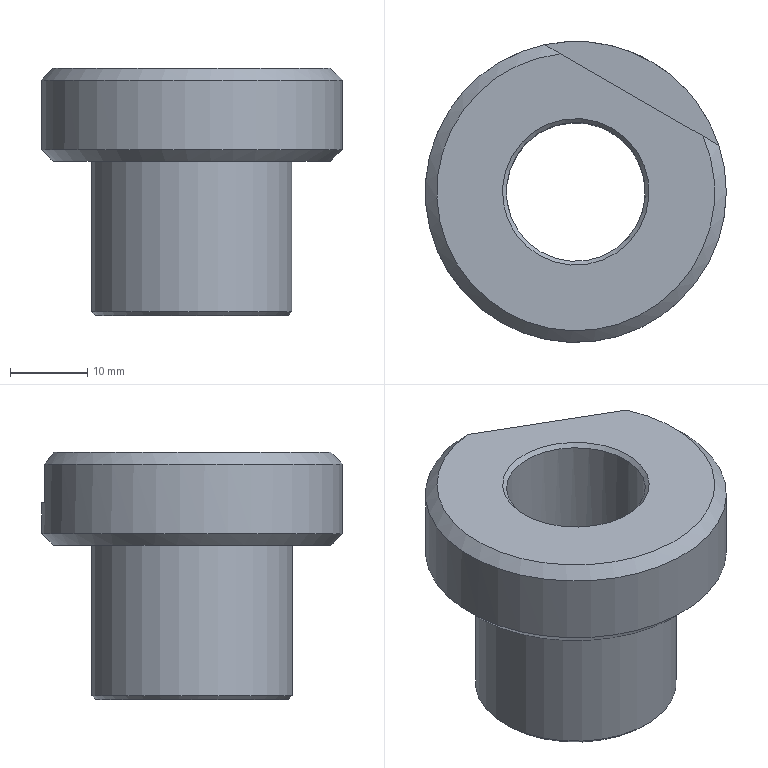Component | NX | DRILL_BUSH | 1 solid | 13 faces | box 39 x 39 x 32 mm | volume 15966 mm3 | plane 5 | cone 5 | cylinder 3 | commonest cylinder face diameters 26 x1 39 x1 18 x1
STEP:
#1=CARTESIAN_POINT('',(0.,0.,0.));
#2=DIRECTION('',(0.,0.,1.));
#3=DIRECTION('',(1.,0.,0.));
#4=AXIS2_PLACEMENT_3D('',#1,#2,#3);
#5=CARTESIAN_POINT('',(-46.25,-80.107,180.));
#6=VERTEX_POINT('',#5);
#7=CARTESIAN_POINT('',(-40.,-69.282,180.));
#8=DIRECTION('',(0.,0.,-1.));
#9=DIRECTION('',(-0.5,-0.866,0.));
#10=AXIS2_PLACEMENT_3D('',#7,#8,#9);
#11=CIRCLE('',#10,12.5);
#12=CARTESIAN_POINT('',(-40.,-69.282,180.));
#13=DIRECTION('',(0.,0.,-1.));
#14=DIRECTION('',(-0.5,-0.866,0.));
#15=AXIS2_PLACEMENT_3D('',#12,#13,#14);
#16=PLANE('',#15);
#17=CARTESIAN_POINT('',(0.,0.));
#18=DIRECTION('',(1.,0.));
#19=AXIS2_PLACEMENT_2D('',#17,#18);
#20=CIRCLE('',#19,12.5);
#21=(GEOMETRIC_REPRESENTATION_CONTEXT(2)PARAMETRIC_REPRESENTATION_CONTEXT()REPRESENTATION_CONTEXT('',''));
#22=DEFINITIONAL_REPRESENTATION('',(#20),#21);
#23=PCURVE('',#16,#22);
#24=CARTESIAN_POINT('',(-40.,-69.282,180.5));
#25=DIRECTION('',(0.,0.,1.));
#26=DIRECTION('',(0.5,0.866,0.));
#27=AXIS2_PLACEMENT_3D('',#24,#25,#26);
#28=CONICAL_SURFACE('',#27,13.,0.7854);
#29=CARTESIAN_POINT('',(9.425,-0.5));
#30=DIRECTION('',(-1.,0.));
#31=VECTOR('',#30,1.);
#32=LINE('',#29,#31);
#33=(GEOMETRIC_REPRESENTATION_CONTEXT(2)PARAMETRIC_REPRESENTATION_CONTEXT()REPRESENTATION_CONTEXT('',''));
#34=DEFINITIONAL_REPRESENTATION('',(#32),#33);
#35=PCURVE('',#28,#34);
#36=SURFACE_CURVE('',#11,(#23,#35),.PCURVE_S1.);
#37=EDGE_CURVE('',#6,#6,#36,.T.);
#38=ORIENTED_EDGE('',*,*,#37,.T.);
#39=EDGE_LOOP('',(#38));
#40=FACE_BOUND('',#39,.T.);
#41=CARTESIAN_POINT('',(-44.75,-77.509,180.));
#42=VERTEX_POINT('',#41);
#43=CARTESIAN_POINT('',(-40.,-69.282,180.));
#44=DIRECTION('',(0.,0.,1.));
#45=DIRECTION('',(-0.5,-0.866,0.));
#46=AXIS2_PLACEMENT_3D('',#43,#44,#45);
#47=CIRCLE('',#46,9.5);
#48=CARTESIAN_POINT('',(9.5,0.));
#49=CARTESIAN_POINT('',(9.5,-16.454));
#50=CARTESIAN_POINT('',(-4.75,-8.227));
#51=CARTESIAN_POINT('',(-19.,-0.));
#52=CARTESIAN_POINT('',(-4.75,8.227));
#53=CARTESIAN_POINT('',(9.5,16.454));
#54=CARTESIAN_POINT('',(9.5,0.));
#55=(BOUNDED_CURVE()B_SPLINE_CURVE(2,(#48,#49,#50,#51,#52,#53,#54),.UNSPECIFIED.,.T.,.F.)B_SPLINE_CURVE_WITH_KNOTS((1,2,2,2,2,1),(-2.094,0.,2.094,4.189,6.283,8.378),.UNSPECIFIED.)CURVE()GEOMETRIC_REPRESENTATION_ITEM()RATIONAL_B_SPLINE_CURVE((1.,0.5,1.,0.5,1.,0.5,1.))REPRESENTATION_ITEM(''));
#56=(GEOMETRIC_REPRESENTATION_CONTEXT(2)PARAMETRIC_REPRESENTATION_CONTEXT()REPRESENTATION_CONTEXT('',''));
#57=DEFINITIONAL_REPRESENTATION('',(#55),#56);
#58=PCURVE('',#16,#57);
#59=CARTESIAN_POINT('',(-40.,-69.282,180.5));
#60=DIRECTION('',(0.,0.,-1.));
#61=DIRECTION('',(-0.5,-0.866,0.));
#62=AXIS2_PLACEMENT_3D('',#59,#60,#61);
#63=CONICAL_SURFACE('',#62,9.,0.7854);
#64=CARTESIAN_POINT('',(6.283,0.5));
#65=DIRECTION('',(-1.,0.));
#66=VECTOR('',#65,1.);
#67=LINE('',#64,#66);
#68=(GEOMETRIC_REPRESENTATION_CONTEXT(2)PARAMETRIC_REPRESENTATION_CONTEXT()REPRESENTATION_CONTEXT('',''));
#69=DEFINITIONAL_REPRESENTATION('',(#67),#68);
#70=PCURVE('',#63,#69);
#71=SURFACE_CURVE('',#47,(#58,#70),.PCURVE_S1.);
#72=EDGE_CURVE('',#42,#42,#71,.T.);
#73=ORIENTED_EDGE('',*,*,#72,.T.);
#74=EDGE_LOOP('',(#73));
#75=FACE_BOUND('',#74,.T.);
#76=ADVANCED_FACE('',(#40,#75),#16,.T.);
#77=CARTESIAN_POINT('',(-46.5,-80.54,180.5));
#78=VERTEX_POINT('',#77);
#79=CARTESIAN_POINT('',(-40.,-69.282,180.5));
#80=DIRECTION('',(0.,0.,1.));
#81=DIRECTION('',(-0.5,-0.866,0.));
#82=AXIS2_PLACEMENT_3D('',#79,#80,#81);
#83=CIRCLE('',#82,13.);
#84=CARTESIAN_POINT('',(-40.,-69.282,180.));
#85=DIRECTION('',(0.,0.,1.));
#86=DIRECTION('',(0.5,0.866,0.));
#87=AXIS2_PLACEMENT_3D('',#84,#85,#86);
#88=CYLINDRICAL_SURFACE('',#87,13.);
#89=CARTESIAN_POINT('',(3.142,0.5));
#90=DIRECTION('',(1.,0.));
#91=VECTOR('',#90,1.);
#92=LINE('',#89,#91);
#93=(GEOMETRIC_REPRESENTATION_CONTEXT(2)PARAMETRIC_REPRESENTATION_CONTEXT()REPRESENTATION_CONTEXT('',''));
#94=DEFINITIONAL_REPRESENTATION('',(#92),#93);
#95=PCURVE('',#88,#94);
#96=CARTESIAN_POINT('',(3.142,0.));
#97=DIRECTION('',(1.,0.));
#98=VECTOR('',#97,1.);
#99=LINE('',#96,#98);
#100=(GEOMETRIC_REPRESENTATION_CONTEXT(2)PARAMETRIC_REPRESENTATION_CONTEXT()REPRESENTATION_CONTEXT('',''));
#101=DEFINITIONAL_REPRESENTATION('',(#99),#100);
#102=PCURVE('',#28,#101);
#103=SURFACE_CURVE('',#83,(#95,#102),.PCURVE_S1.);
#104=EDGE_CURVE('',#78,#78,#103,.T.);
#105=ORIENTED_EDGE('',*,*,#104,.T.);
#106=CARTESIAN_POINT('',(-46.5,-80.54,200.));
#107=VERTEX_POINT('',#106);
#108=CARTESIAN_POINT('',(-46.5,-80.54,180.5));
#109=CARTESIAN_POINT('',(-46.5,-80.54,200.));
#110=B_SPLINE_CURVE_WITH_KNOTS('',1,(#108,#109),.UNSPECIFIED.,.F.,.F.,(2,2),(0.5,20.),.PIECEWISE_BEZIER_KNOTS.);
#111=CARTESIAN_POINT('',(9.425,0.));
#112=DIRECTION('',(0.,1.));
#113=VECTOR('',#112,1.);
#114=LINE('',#111,#113);
#115=(GEOMETRIC_REPRESENTATION_CONTEXT(2)PARAMETRIC_REPRESENTATION_CONTEXT()REPRESENTATION_CONTEXT('',''));
#116=DEFINITIONAL_REPRESENTATION('',(#114),#115);
#117=PCURVE('',#88,#116);
#118=CARTESIAN_POINT('',(3.142,0.));
#119=DIRECTION('',(0.,1.));
#120=VECTOR('',#119,1.);
#121=LINE('',#118,#120);
#122=(GEOMETRIC_REPRESENTATION_CONTEXT(2)PARAMETRIC_REPRESENTATION_CONTEXT()REPRESENTATION_CONTEXT('',''));
#123=DEFINITIONAL_REPRESENTATION('',(#121),#122);
#124=PCURVE('',#88,#123);
#125=SEAM_CURVE('',#110,(#117,#124),.PCURVE_S1.);
#126=EDGE_CURVE('',#78,#107,#125,.T.);
#127=ORIENTED_EDGE('',*,*,#126,.T.);
#128=CARTESIAN_POINT('',(-40.,-69.282,200.));
#129=DIRECTION('',(0.,0.,1.));
#130=DIRECTION('',(-0.5,-0.866,0.));
#131=AXIS2_PLACEMENT_3D('',#128,#129,#130);
#132=CIRCLE('',#131,13.);
#133=CARTESIAN_POINT('',(3.142,20.));
#134=DIRECTION('',(1.,0.));
#135=VECTOR('',#134,1.);
#136=LINE('',#133,#135);
#137=(GEOMETRIC_REPRESENTATION_CONTEXT(2)PARAMETRIC_REPRESENTATION_CONTEXT()REPRESENTATION_CONTEXT('',''));
#138=DEFINITIONAL_REPRESENTATION('',(#136),#137);
#139=PCURVE('',#88,#138);
#140=CARTESIAN_POINT('',(-40.,-69.282,200.));
#141=DIRECTION('',(0.,0.,-1.));
#142=DIRECTION('',(-0.5,-0.866,0.));
#143=AXIS2_PLACEMENT_3D('',#140,#141,#142);
#144=PLANE('',#143);
#145=CARTESIAN_POINT('',(13.,0.));
#146=CARTESIAN_POINT('',(13.,-22.517));
#147=CARTESIAN_POINT('',(-6.5,-11.258));
#148=CARTESIAN_POINT('',(-26.,-0.));
#149=CARTESIAN_POINT('',(-6.5,11.258));
#150=CARTESIAN_POINT('',(13.,22.517));
#151=CARTESIAN_POINT('',(13.,0.));
#152=(BOUNDED_CURVE()B_SPLINE_CURVE(2,(#145,#146,#147,#148,#149,#150,#151),.UNSPECIFIED.,.T.,.F.)B_SPLINE_CURVE_WITH_KNOTS((1,2,2,2,2,1),(-2.094,0.,2.094,4.189,6.283,8.378),.UNSPECIFIED.)CURVE()GEOMETRIC_REPRESENTATION_ITEM()RATIONAL_B_SPLINE_CURVE((1.,0.5,1.,0.5,1.,0.5,1.))REPRESENTATION_ITEM(''));
#153=(GEOMETRIC_REPRESENTATION_CONTEXT(2)PARAMETRIC_REPRESENTATION_CONTEXT()REPRESENTATION_CONTEXT('',''));
#154=DEFINITIONAL_REPRESENTATION('',(#152),#153);
#155=PCURVE('',#144,#154);
#156=SURFACE_CURVE('',#132,(#139,#155),.PCURVE_S1.);
#157=EDGE_CURVE('',#107,#107,#156,.T.);
#158=ORIENTED_EDGE('',*,*,#157,.F.);
#159=ORIENTED_EDGE('',*,*,#126,.F.);
#160=EDGE_LOOP('',(#105,#127,#158,#159));
#161=FACE_BOUND('',#160,.T.);
#162=ADVANCED_FACE('',(#161),#88,.T.);
#163=CARTESIAN_POINT('',(-35.25,-61.055,212.));
#164=VERTEX_POINT('',#163);
#165=CARTESIAN_POINT('',(-40.,-69.282,212.));
#166=DIRECTION('',(0.,0.,-1.));
#167=DIRECTION('',(0.5,0.866,0.));
#168=AXIS2_PLACEMENT_3D('',#165,#166,#167);
#169=CIRCLE('',#168,9.5);
#170=CARTESIAN_POINT('',(-40.,-69.282,212.));
#171=DIRECTION('',(0.,0.,1.));
#172=DIRECTION('',(0.5,0.866,0.));
#173=AXIS2_PLACEMENT_3D('',#170,#171,#172);
#174=PLANE('',#173);
#175=CARTESIAN_POINT('',(9.5,0.));
#176=CARTESIAN_POINT('',(9.5,-16.454));
#177=CARTESIAN_POINT('',(-4.75,-8.227));
#178=CARTESIAN_POINT('',(-19.,-0.));
#179=CARTESIAN_POINT('',(-4.75,8.227));
#180=CARTESIAN_POINT('',(9.5,16.454));
#181=CARTESIAN_POINT('',(9.5,0.));
#182=(BOUNDED_CURVE()B_SPLINE_CURVE(2,(#175,#176,#177,#178,#179,#180,#181),.UNSPECIFIED.,.T.,.F.)B_SPLINE_CURVE_WITH_KNOTS((1,2,2,2,2,1),(-2.094,0.,2.094,4.189,6.283,8.378),.UNSPECIFIED.)CURVE()GEOMETRIC_REPRESENTATION_ITEM()RATIONAL_B_SPLINE_CURVE((1.,0.5,1.,0.5,1.,0.5,1.))REPRESENTATION_ITEM(''));
#183=(GEOMETRIC_REPRESENTATION_CONTEXT(2)PARAMETRIC_REPRESENTATION_CONTEXT()REPRESENTATION_CONTEXT('',''));
#184=DEFINITIONAL_REPRESENTATION('',(#182),#183);
#185=PCURVE('',#174,#184);
#186=CARTESIAN_POINT('',(-40.,-69.282,212.));
#187=DIRECTION('',(0.,0.,1.));
#188=DIRECTION('',(0.5,0.866,0.));
#189=AXIS2_PLACEMENT_3D('',#186,#187,#188);
#190=CONICAL_SURFACE('',#189,9.5,0.7854);
#191=CARTESIAN_POINT('',(6.283,0.));
#192=DIRECTION('',(-1.,0.));
#193=VECTOR('',#192,1.);
#194=LINE('',#191,#193);
#195=(GEOMETRIC_REPRESENTATION_CONTEXT(2)PARAMETRIC_REPRESENTATION_CONTEXT()REPRESENTATION_CONTEXT('',''));
#196=DEFINITIONAL_REPRESENTATION('',(#194),#195);
#197=PCURVE('',#190,#196);
#198=SURFACE_CURVE('',#169,(#185,#197),.PCURVE_S1.);
#199=EDGE_CURVE('',#164,#164,#198,.T.);
#200=ORIENTED_EDGE('',*,*,#199,.T.);
#201=EDGE_LOOP('',(#200));
#202=FACE_BOUND('',#201,.T.);
#203=CARTESIAN_POINT('',(-41.986,-51.392,212.));
#204=VERTEX_POINT('',#203);
#205=CARTESIAN_POINT('',(-23.514,-62.057,212.));
#206=VERTEX_POINT('',#205);
#207=CARTESIAN_POINT('',(-52.669,-45.225,212.));
#208=DIRECTION('',(0.866,-0.5,0.));
#209=VECTOR('',#208,1.);
#210=LINE('',#207,#209);
#211=CARTESIAN_POINT('',(14.5,23.));
#212=DIRECTION('',(0.,-1.));
#213=VECTOR('',#212,1.);
#214=LINE('',#211,#213);
#215=(GEOMETRIC_REPRESENTATION_CONTEXT(2)PARAMETRIC_REPRESENTATION_CONTEXT()REPRESENTATION_CONTEXT('',''));
#216=DEFINITIONAL_REPRESENTATION('',(#214),#215);
#217=PCURVE('',#174,#216);
#218=CARTESIAN_POINT('',(-52.669,-45.225,205.5));
#219=DIRECTION('',(-0.5,-0.866,0.));
#220=DIRECTION('',(0.866,-0.5,0.));
#221=AXIS2_PLACEMENT_3D('',#218,#219,#220);
#222=PLANE('',#221);
#223=CARTESIAN_POINT('',(0.,6.5));
#224=DIRECTION('',(1.,0.));
#225=VECTOR('',#224,1.);
#226=LINE('',#223,#225);
#227=(GEOMETRIC_REPRESENTATION_CONTEXT(2)PARAMETRIC_REPRESENTATION_CONTEXT()REPRESENTATION_CONTEXT('',''));
#228=DEFINITIONAL_REPRESENTATION('',(#226),#227);
#229=PCURVE('',#222,#228);
#230=SURFACE_CURVE('',#210,(#217,#229),.PCURVE_S1.);
#231=EDGE_CURVE('',#204,#206,#230,.T.);
#232=ORIENTED_EDGE('',*,*,#231,.F.);
#233=CARTESIAN_POINT('',(-40.,-69.282,212.));
#234=DIRECTION('',(0.,0.,1.));
#235=DIRECTION('',(0.5,0.866,0.));
#236=AXIS2_PLACEMENT_3D('',#233,#234,#235);
#237=CIRCLE('',#236,18.);
#238=CARTESIAN_POINT('',(0.,0.));
#239=DIRECTION('',(1.,0.));
#240=AXIS2_PLACEMENT_2D('',#238,#239);
#241=CIRCLE('',#240,18.);
#242=(GEOMETRIC_REPRESENTATION_CONTEXT(2)PARAMETRIC_REPRESENTATION_CONTEXT()REPRESENTATION_CONTEXT('',''));
#243=DEFINITIONAL_REPRESENTATION('',(#241),#242);
#244=PCURVE('',#174,#243);
#245=CARTESIAN_POINT('',(-40.,-69.282,210.5));
#246=DIRECTION('',(0.,0.,-1.));
#247=DIRECTION('',(-0.5,-0.866,0.));
#248=AXIS2_PLACEMENT_3D('',#245,#246,#247);
#249=CONICAL_SURFACE('',#248,19.5,0.7854);
#250=CARTESIAN_POINT('',(9.425,-1.5));
#251=DIRECTION('',(-1.,0.));
#252=VECTOR('',#251,1.);
#253=LINE('',#250,#252);
#254=(GEOMETRIC_REPRESENTATION_CONTEXT(2)PARAMETRIC_REPRESENTATION_CONTEXT()REPRESENTATION_CONTEXT('',''));
#255=DEFINITIONAL_REPRESENTATION('',(#253),#254);
#256=PCURVE('',#249,#255);
#257=SURFACE_CURVE('',#237,(#244,#256),.PCURVE_S1.);
#258=EDGE_CURVE('',#204,#206,#257,.T.);
#259=ORIENTED_EDGE('',*,*,#258,.T.);
#260=EDGE_LOOP('',(#232,#259));
#261=FACE_BOUND('',#260,.T.);
#262=ADVANCED_FACE('',(#202,#261),#174,.T.);
#263=CARTESIAN_POINT('',(-49.,-84.87,200.));
#264=VERTEX_POINT('',#263);
#265=CARTESIAN_POINT('',(-40.,-69.282,200.));
#266=DIRECTION('',(0.,0.,-1.));
#267=DIRECTION('',(-0.5,-0.866,0.));
#268=AXIS2_PLACEMENT_3D('',#265,#266,#267);
#269=CIRCLE('',#268,18.);
#270=CARTESIAN_POINT('',(0.,0.));
#271=DIRECTION('',(1.,0.));
#272=AXIS2_PLACEMENT_2D('',#270,#271);
#273=CIRCLE('',#272,18.);
#274=(GEOMETRIC_REPRESENTATION_CONTEXT(2)PARAMETRIC_REPRESENTATION_CONTEXT()REPRESENTATION_CONTEXT('',''));
#275=DEFINITIONAL_REPRESENTATION('',(#273),#274);
#276=PCURVE('',#144,#275);
#277=CARTESIAN_POINT('',(-40.,-69.282,201.5));
#278=DIRECTION('',(0.,0.,1.));
#279=DIRECTION('',(0.5,0.866,0.));
#280=AXIS2_PLACEMENT_3D('',#277,#278,#279);
#281=CONICAL_SURFACE('',#280,19.5,0.7854);
#282=CARTESIAN_POINT('',(9.425,-1.5));
#283=DIRECTION('',(-1.,0.));
#284=VECTOR('',#283,1.);
#285=LINE('',#282,#284);
#286=(GEOMETRIC_REPRESENTATION_CONTEXT(2)PARAMETRIC_REPRESENTATION_CONTEXT()REPRESENTATION_CONTEXT('',''));
#287=DEFINITIONAL_REPRESENTATION('',(#285),#286);
#288=PCURVE('',#281,#287);
#289=SURFACE_CURVE('',#269,(#276,#288),.PCURVE_S1.);
#290=EDGE_CURVE('',#264,#264,#289,.T.);
#291=ORIENTED_EDGE('',*,*,#290,.T.);
#292=EDGE_LOOP('',(#291));
#293=FACE_BOUND('',#292,.T.);
#294=ORIENTED_EDGE('',*,*,#157,.T.);
#295=EDGE_LOOP('',(#294));
#296=FACE_BOUND('',#295,.T.);
#297=ADVANCED_FACE('',(#293,#296),#144,.T.);
#298=CARTESIAN_POINT('',(-49.75,-86.17,201.5));
#299=VERTEX_POINT('',#298);
#300=CARTESIAN_POINT('',(-21.458,-63.244,201.5));
#301=VERTEX_POINT('',#300);
#302=CARTESIAN_POINT('',(-40.,-69.282,201.5));
#303=DIRECTION('',(0.,0.,1.));
#304=DIRECTION('',(-0.5,-0.866,0.));
#305=AXIS2_PLACEMENT_3D('',#302,#303,#304);
#306=CIRCLE('',#305,19.5);
#307=CARTESIAN_POINT('',(-40.,-69.282,200.));
#308=DIRECTION('',(0.,0.,1.));
#309=DIRECTION('',(0.5,0.866,0.));
#310=AXIS2_PLACEMENT_3D('',#307,#308,#309);
#311=CYLINDRICAL_SURFACE('',#310,19.5);
#312=CARTESIAN_POINT('',(9.425,1.5));
#313=DIRECTION('',(1.,0.));
#314=VECTOR('',#313,1.);
#315=LINE('',#312,#314);
#316=(GEOMETRIC_REPRESENTATION_CONTEXT(2)PARAMETRIC_REPRESENTATION_CONTEXT()REPRESENTATION_CONTEXT('',''));
#317=DEFINITIONAL_REPRESENTATION('',(#315),#316);
#318=PCURVE('',#311,#317);
#319=CARTESIAN_POINT('',(3.142,0.));
#320=DIRECTION('',(1.,-0.));
#321=VECTOR('',#320,1.);
#322=LINE('',#319,#321);
#323=(GEOMETRIC_REPRESENTATION_CONTEXT(2)PARAMETRIC_REPRESENTATION_CONTEXT()REPRESENTATION_CONTEXT('',''));
#324=DEFINITIONAL_REPRESENTATION('',(#322),#323);
#325=PCURVE('',#281,#324);
#326=SURFACE_CURVE('',#306,(#318,#325),.PCURVE_S1.);
#327=EDGE_CURVE('',#299,#301,#326,.T.);
#328=ORIENTED_EDGE('',*,*,#327,.T.);
#329=CARTESIAN_POINT('',(-21.458,-63.244,205.5));
#330=VERTEX_POINT('',#329);
#331=CARTESIAN_POINT('',(-21.458,-63.244,201.5));
#332=CARTESIAN_POINT('',(-21.458,-63.244,205.5));
#333=B_SPLINE_CURVE_WITH_KNOTS('',1,(#331,#332),.UNSPECIFIED.,.F.,.F.,(2,2),(1.5,5.5),.PIECEWISE_BEZIER_KNOTS.);
#334=CARTESIAN_POINT('',(11.834,0.));
#335=DIRECTION('',(0.,1.));
#336=VECTOR('',#335,1.);
#337=LINE('',#334,#336);
#338=(GEOMETRIC_REPRESENTATION_CONTEXT(2)PARAMETRIC_REPRESENTATION_CONTEXT()REPRESENTATION_CONTEXT('',''));
#339=DEFINITIONAL_REPRESENTATION('',(#337),#338);
#340=PCURVE('',#311,#339);
#341=CARTESIAN_POINT('',(5.551,0.));
#342=DIRECTION('',(0.,1.));
#343=VECTOR('',#342,1.);
#344=LINE('',#341,#343);
#345=(GEOMETRIC_REPRESENTATION_CONTEXT(2)PARAMETRIC_REPRESENTATION_CONTEXT()REPRESENTATION_CONTEXT('',''));
#346=DEFINITIONAL_REPRESENTATION('',(#344),#345);
#347=PCURVE('',#311,#346);
#348=SEAM_CURVE('',#333,(#340,#347),.PCURVE_S1.);
#349=EDGE_CURVE('',#301,#330,#348,.T.);
#350=ORIENTED_EDGE('',*,*,#349,.T.);
#351=CARTESIAN_POINT('',(-21.458,-63.244,210.5));
#352=VERTEX_POINT('',#351);
#353=CARTESIAN_POINT('',(-21.458,-63.244,200.));
#354=DIRECTION('',(0.,0.,-1.));
#355=VECTOR('',#354,1.);
#356=LINE('',#353,#355);
#357=CARTESIAN_POINT('',(11.834,0.));
#358=DIRECTION('',(0.,-1.));
#359=VECTOR('',#358,1.);
#360=LINE('',#357,#359);
#361=(GEOMETRIC_REPRESENTATION_CONTEXT(2)PARAMETRIC_REPRESENTATION_CONTEXT()REPRESENTATION_CONTEXT('',''));
#362=DEFINITIONAL_REPRESENTATION('',(#360),#361);
#363=PCURVE('',#311,#362);
#364=CARTESIAN_POINT('',(36.038,-5.5));
#365=DIRECTION('',(0.,-1.));
#366=VECTOR('',#365,1.);
#367=LINE('',#364,#366);
#368=(GEOMETRIC_REPRESENTATION_CONTEXT(2)PARAMETRIC_REPRESENTATION_CONTEXT()REPRESENTATION_CONTEXT('',''));
#369=DEFINITIONAL_REPRESENTATION('',(#367),#368);
#370=PCURVE('',#222,#369);
#371=SURFACE_CURVE('',#356,(#363,#370),.PCURVE_S1.);
#372=EDGE_CURVE('',#352,#330,#371,.T.);
#373=ORIENTED_EDGE('',*,*,#372,.F.);
#374=CARTESIAN_POINT('',(-44.042,-50.205,210.5));
#375=VERTEX_POINT('',#374);
#376=CARTESIAN_POINT('',(-40.,-69.282,210.5));
#377=DIRECTION('',(0.,0.,-1.));
#378=DIRECTION('',(0.5,0.866,0.));
#379=AXIS2_PLACEMENT_3D('',#376,#377,#378);
#380=CIRCLE('',#379,19.5);
#381=CARTESIAN_POINT('',(12.566,10.5));
#382=DIRECTION('',(-1.,0.));
#383=VECTOR('',#382,1.);
#384=LINE('',#381,#383);
#385=(GEOMETRIC_REPRESENTATION_CONTEXT(2)PARAMETRIC_REPRESENTATION_CONTEXT()REPRESENTATION_CONTEXT('',''));
#386=DEFINITIONAL_REPRESENTATION('',(#384),#385);
#387=PCURVE('',#311,#386);
#388=CARTESIAN_POINT('',(3.142,0.));
#389=DIRECTION('',(1.,-0.));
#390=VECTOR('',#389,1.);
#391=LINE('',#388,#390);
#392=(GEOMETRIC_REPRESENTATION_CONTEXT(2)PARAMETRIC_REPRESENTATION_CONTEXT()REPRESENTATION_CONTEXT('',''));
#393=DEFINITIONAL_REPRESENTATION('',(#391),#392);
#394=PCURVE('',#249,#393);
#395=SURFACE_CURVE('',#380,(#387,#394),.PCURVE_S1.);
#396=EDGE_CURVE('',#352,#375,#395,.T.);
#397=ORIENTED_EDGE('',*,*,#396,.T.);
#398=CARTESIAN_POINT('',(-44.042,-50.205,205.5));
#399=VERTEX_POINT('',#398);
#400=CARTESIAN_POINT('',(-44.042,-50.205,200.));
#401=DIRECTION('',(0.,0.,1.));
#402=VECTOR('',#401,1.);
#403=LINE('',#400,#402);
#404=CARTESIAN_POINT('',(7.016,0.));
#405=DIRECTION('',(0.,1.));
#406=VECTOR('',#405,1.);
#407=LINE('',#404,#406);
#408=(GEOMETRIC_REPRESENTATION_CONTEXT(2)PARAMETRIC_REPRESENTATION_CONTEXT()REPRESENTATION_CONTEXT('',''));
#409=DEFINITIONAL_REPRESENTATION('',(#407),#408);
#410=PCURVE('',#311,#409);
#411=CARTESIAN_POINT('',(9.962,-5.5));
#412=DIRECTION('',(0.,1.));
#413=VECTOR('',#412,1.);
#414=LINE('',#411,#413);
#415=(GEOMETRIC_REPRESENTATION_CONTEXT(2)PARAMETRIC_REPRESENTATION_CONTEXT()REPRESENTATION_CONTEXT('',''));
#416=DEFINITIONAL_REPRESENTATION('',(#414),#415);
#417=PCURVE('',#222,#416);
#418=SURFACE_CURVE('',#403,(#410,#417),.PCURVE_S1.);
#419=EDGE_CURVE('',#399,#375,#418,.T.);
#420=ORIENTED_EDGE('',*,*,#419,.F.);
#421=CARTESIAN_POINT('',(-40.,-69.282,205.5));
#422=DIRECTION('',(0.,0.,-1.));
#423=DIRECTION('',(0.5,0.866,0.));
#424=AXIS2_PLACEMENT_3D('',#421,#422,#423);
#425=CIRCLE('',#424,19.5);
#426=CARTESIAN_POINT('',(12.566,5.5));
#427=DIRECTION('',(-1.,0.));
#428=VECTOR('',#427,1.);
#429=LINE('',#426,#428);
#430=(GEOMETRIC_REPRESENTATION_CONTEXT(2)PARAMETRIC_REPRESENTATION_CONTEXT()REPRESENTATION_CONTEXT('',''));
#431=DEFINITIONAL_REPRESENTATION('',(#429),#430);
#432=PCURVE('',#311,#431);
#433=CARTESIAN_POINT('',(-40.,-69.282,205.5));
#434=DIRECTION('',(0.,0.,1.));
#435=DIRECTION('',(0.5,0.866,0.));
#436=AXIS2_PLACEMENT_3D('',#433,#434,#435);
#437=PLANE('',#436);
#438=CARTESIAN_POINT('',(19.5,0.));
#439=CARTESIAN_POINT('',(19.5,-33.775));
#440=CARTESIAN_POINT('',(-9.75,-16.887));
#441=CARTESIAN_POINT('',(-39.,-0.));
#442=CARTESIAN_POINT('',(-9.75,16.887));
#443=CARTESIAN_POINT('',(19.5,33.775));
#444=CARTESIAN_POINT('',(19.5,0.));
#445=(BOUNDED_CURVE()B_SPLINE_CURVE(2,(#438,#439,#440,#441,#442,#443,#444),.UNSPECIFIED.,.T.,.F.)B_SPLINE_CURVE_WITH_KNOTS((1,2,2,2,2,1),(-2.094,0.,2.094,4.189,6.283,8.378),.UNSPECIFIED.)CURVE()GEOMETRIC_REPRESENTATION_ITEM()RATIONAL_B_SPLINE_CURVE((1.,0.5,1.,0.5,1.,0.5,1.))REPRESENTATION_ITEM(''));
#446=(GEOMETRIC_REPRESENTATION_CONTEXT(2)PARAMETRIC_REPRESENTATION_CONTEXT()REPRESENTATION_CONTEXT('',''));
#447=DEFINITIONAL_REPRESENTATION('',(#445),#446);
#448=PCURVE('',#437,#447);
#449=SURFACE_CURVE('',#425,(#432,#448),.PCURVE_S1.);
#450=EDGE_CURVE('',#399,#330,#449,.T.);
#451=ORIENTED_EDGE('',*,*,#450,.T.);
#452=ORIENTED_EDGE('',*,*,#349,.F.);
#453=CARTESIAN_POINT('',(-40.,-69.282,201.5));
#454=DIRECTION('',(0.,0.,1.));
#455=DIRECTION('',(-0.5,-0.866,0.));
#456=AXIS2_PLACEMENT_3D('',#453,#454,#455);
#457=CIRCLE('',#456,19.5);
#458=CARTESIAN_POINT('',(3.142,1.5));
#459=DIRECTION('',(1.,0.));
#460=VECTOR('',#459,1.);
#461=LINE('',#458,#460);
#462=(GEOMETRIC_REPRESENTATION_CONTEXT(2)PARAMETRIC_REPRESENTATION_CONTEXT()REPRESENTATION_CONTEXT('',''));
#463=DEFINITIONAL_REPRESENTATION('',(#461),#462);
#464=PCURVE('',#311,#463);
#465=CARTESIAN_POINT('',(3.142,-0.));
#466=DIRECTION('',(1.,0.));
#467=VECTOR('',#466,1.);
#468=LINE('',#465,#467);
#469=(GEOMETRIC_REPRESENTATION_CONTEXT(2)PARAMETRIC_REPRESENTATION_CONTEXT()REPRESENTATION_CONTEXT('',''));
#470=DEFINITIONAL_REPRESENTATION('',(#468),#469);
#471=PCURVE('',#281,#470);
#472=SURFACE_CURVE('',#457,(#464,#471),.PCURVE_S1.);
#473=EDGE_CURVE('',#301,#299,#472,.T.);
#474=ORIENTED_EDGE('',*,*,#473,.T.);
#475=EDGE_LOOP('',(#328,#350,#373,#397,#420,#451,#452,#474));
#476=FACE_BOUND('',#475,.T.);
#477=ADVANCED_FACE('',(#476),#311,.T.);
#478=CARTESIAN_POINT('',(-44.5,-77.076,180.5));
#479=VERTEX_POINT('',#478);
#480=CARTESIAN_POINT('',(-40.,-69.282,180.5));
#481=DIRECTION('',(0.,0.,-1.));
#482=DIRECTION('',(-0.5,-0.866,0.));
#483=AXIS2_PLACEMENT_3D('',#480,#481,#482);
#484=CIRCLE('',#483,9.);
#485=CARTESIAN_POINT('',(-40.,-69.282,212.));
#486=DIRECTION('',(0.,0.,-1.));
#487=DIRECTION('',(-0.5,-0.866,0.));
#488=AXIS2_PLACEMENT_3D('',#485,#486,#487);
#489=CYLINDRICAL_SURFACE('',#488,9.);
#490=CARTESIAN_POINT('',(0.,31.5));
#491=DIRECTION('',(1.,0.));
#492=VECTOR('',#491,1.);
#493=LINE('',#490,#492);
#494=(GEOMETRIC_REPRESENTATION_CONTEXT(2)PARAMETRIC_REPRESENTATION_CONTEXT()REPRESENTATION_CONTEXT('',''));
#495=DEFINITIONAL_REPRESENTATION('',(#493),#494);
#496=PCURVE('',#489,#495);
#497=CARTESIAN_POINT('',(0.,0.));
#498=DIRECTION('',(1.,0.));
#499=VECTOR('',#498,1.);
#500=LINE('',#497,#499);
#501=(GEOMETRIC_REPRESENTATION_CONTEXT(2)PARAMETRIC_REPRESENTATION_CONTEXT()REPRESENTATION_CONTEXT('',''));
#502=DEFINITIONAL_REPRESENTATION('',(#500),#501);
#503=PCURVE('',#63,#502);
#504=SURFACE_CURVE('',#484,(#496,#503),.PCURVE_S1.);
#505=EDGE_CURVE('',#479,#479,#504,.T.);
#506=ORIENTED_EDGE('',*,*,#505,.F.);
#507=CARTESIAN_POINT('',(-44.5,-77.076,211.5));
#508=VERTEX_POINT('',#507);
#509=CARTESIAN_POINT('',(-44.5,-77.076,211.5));
#510=CARTESIAN_POINT('',(-44.5,-77.076,180.5));
#511=B_SPLINE_CURVE_WITH_KNOTS('',1,(#509,#510),.UNSPECIFIED.,.F.,.F.,(2,2),(0.5,31.5),.PIECEWISE_BEZIER_KNOTS.);
#512=CARTESIAN_POINT('',(0.,0.));
#513=DIRECTION('',(0.,1.));
#514=VECTOR('',#513,1.);
#515=LINE('',#512,#514);
#516=(GEOMETRIC_REPRESENTATION_CONTEXT(2)PARAMETRIC_REPRESENTATION_CONTEXT()REPRESENTATION_CONTEXT('',''));
#517=DEFINITIONAL_REPRESENTATION('',(#515),#516);
#518=PCURVE('',#489,#517);
#519=CARTESIAN_POINT('',(6.283,0.));
#520=DIRECTION('',(0.,1.));
#521=VECTOR('',#520,1.);
#522=LINE('',#519,#521);
#523=(GEOMETRIC_REPRESENTATION_CONTEXT(2)PARAMETRIC_REPRESENTATION_CONTEXT()REPRESENTATION_CONTEXT('',''));
#524=DEFINITIONAL_REPRESENTATION('',(#522),#523);
#525=PCURVE('',#489,#524);
#526=SEAM_CURVE('',#511,(#518,#525),.PCURVE_S1.);
#527=EDGE_CURVE('',#508,#479,#526,.T.);
#528=ORIENTED_EDGE('',*,*,#527,.F.);
#529=CARTESIAN_POINT('',(-35.5,-61.488,211.5));
#530=VERTEX_POINT('',#529);
#531=CARTESIAN_POINT('',(-40.,-69.282,211.5));
#532=DIRECTION('',(0.,0.,1.));
#533=DIRECTION('',(0.5,0.866,0.));
#534=AXIS2_PLACEMENT_3D('',#531,#532,#533);
#535=CIRCLE('',#534,9.);
#536=CARTESIAN_POINT('',(3.142,0.5));
#537=DIRECTION('',(-1.,0.));
#538=VECTOR('',#537,1.);
#539=LINE('',#536,#538);
#540=(GEOMETRIC_REPRESENTATION_CONTEXT(2)PARAMETRIC_REPRESENTATION_CONTEXT()REPRESENTATION_CONTEXT('',''));
#541=DEFINITIONAL_REPRESENTATION('',(#539),#540);
#542=PCURVE('',#489,#541);
#543=CARTESIAN_POINT('',(0.,-0.5));
#544=DIRECTION('',(1.,0.));
#545=VECTOR('',#544,1.);
#546=LINE('',#543,#545);
#547=(GEOMETRIC_REPRESENTATION_CONTEXT(2)PARAMETRIC_REPRESENTATION_CONTEXT()REPRESENTATION_CONTEXT('',''));
#548=DEFINITIONAL_REPRESENTATION('',(#546),#547);
#549=PCURVE('',#190,#548);
#550=SURFACE_CURVE('',#535,(#542,#549),.PCURVE_S1.);
#551=EDGE_CURVE('',#530,#508,#550,.T.);
#552=ORIENTED_EDGE('',*,*,#551,.F.);
#553=CARTESIAN_POINT('',(-40.,-69.282,211.5));
#554=DIRECTION('',(0.,0.,1.));
#555=DIRECTION('',(0.5,0.866,0.));
#556=AXIS2_PLACEMENT_3D('',#553,#554,#555);
#557=CIRCLE('',#556,9.);
#558=CARTESIAN_POINT('',(9.425,0.5));
#559=DIRECTION('',(-1.,0.));
#560=VECTOR('',#559,1.);
#561=LINE('',#558,#560);
#562=(GEOMETRIC_REPRESENTATION_CONTEXT(2)PARAMETRIC_REPRESENTATION_CONTEXT()REPRESENTATION_CONTEXT('',''));
#563=DEFINITIONAL_REPRESENTATION('',(#561),#562);
#564=PCURVE('',#489,#563);
#565=CARTESIAN_POINT('',(-0.,-0.5));
#566=DIRECTION('',(1.,0.));
#567=VECTOR('',#566,1.);
#568=LINE('',#565,#567);
#569=(GEOMETRIC_REPRESENTATION_CONTEXT(2)PARAMETRIC_REPRESENTATION_CONTEXT()REPRESENTATION_CONTEXT('',''));
#570=DEFINITIONAL_REPRESENTATION('',(#568),#569);
#571=PCURVE('',#190,#570);
#572=SURFACE_CURVE('',#557,(#564,#571),.PCURVE_S1.);
#573=EDGE_CURVE('',#508,#530,#572,.T.);
#574=ORIENTED_EDGE('',*,*,#573,.F.);
#575=ORIENTED_EDGE('',*,*,#527,.T.);
#576=EDGE_LOOP('',(#506,#528,#552,#574,#575));
#577=FACE_BOUND('',#576,.F.);
#578=ADVANCED_FACE('',(#577),#489,.F.);
#579=ORIENTED_EDGE('',*,*,#419,.T.);
#580=CARTESIAN_POINT('',(-44.042,-50.205,210.5));
#581=CARTESIAN_POINT('',(-43.368,-50.594,211.02));
#582=CARTESIAN_POINT('',(-42.684,-50.989,211.523));
#583=CARTESIAN_POINT('',(-41.986,-51.392,212.));
#584=B_SPLINE_CURVE_WITH_KNOTS('',3,(#580,#581,#582,#583),.UNSPECIFIED.,.F.,.F.,(4,4),(0.,1.),.PIECEWISE_BEZIER_KNOTS.);
#585=CARTESIAN_POINT('',(9.962,5.));
#586=CARTESIAN_POINT('',(10.74,5.52));
#587=CARTESIAN_POINT('',(11.53,6.023));
#588=CARTESIAN_POINT('',(12.335,6.5));
#589=B_SPLINE_CURVE_WITH_KNOTS('',3,(#585,#586,#587,#588),.UNSPECIFIED.,.F.,.F.,(4,4),(0.,1.),.PIECEWISE_BEZIER_KNOTS.);
#590=(GEOMETRIC_REPRESENTATION_CONTEXT(2)PARAMETRIC_REPRESENTATION_CONTEXT()REPRESENTATION_CONTEXT('',''));
#591=DEFINITIONAL_REPRESENTATION('',(#589),#590);
#592=PCURVE('',#222,#591);
#593=CARTESIAN_POINT('',(8.692,0.));
#594=CARTESIAN_POINT('',(8.791,-1.5));
#595=B_SPLINE_CURVE_WITH_KNOTS('',1,(#593,#594),.UNSPECIFIED.,.F.,.F.,(2,2),(0.,1.),.PIECEWISE_BEZIER_KNOTS.);
#596=(GEOMETRIC_REPRESENTATION_CONTEXT(2)PARAMETRIC_REPRESENTATION_CONTEXT()REPRESENTATION_CONTEXT('',''));
#597=DEFINITIONAL_REPRESENTATION('',(#595),#596);
#598=PCURVE('',#249,#597);
#599=SURFACE_CURVE('',#584,(#592,#598),.PCURVE_S1.);
#600=EDGE_CURVE('',#375,#204,#599,.T.);
#601=ORIENTED_EDGE('',*,*,#600,.T.);
#602=ORIENTED_EDGE('',*,*,#231,.T.);
#603=CARTESIAN_POINT('',(-23.514,-62.057,212.));
#604=CARTESIAN_POINT('',(-22.816,-62.46,211.523));
#605=CARTESIAN_POINT('',(-22.132,-62.855,211.02));
#606=CARTESIAN_POINT('',(-21.458,-63.244,210.5));
#607=B_SPLINE_CURVE_WITH_KNOTS('',3,(#603,#604,#605,#606),.UNSPECIFIED.,.F.,.F.,(4,4),(0.,1.),.PIECEWISE_BEZIER_KNOTS.);
#608=CARTESIAN_POINT('',(33.665,6.5));
#609=CARTESIAN_POINT('',(34.47,6.023));
#610=CARTESIAN_POINT('',(35.26,5.52));
#611=CARTESIAN_POINT('',(36.038,5.));
#612=B_SPLINE_CURVE_WITH_KNOTS('',3,(#608,#609,#610,#611),.UNSPECIFIED.,.F.,.F.,(4,4),(0.,1.),.PIECEWISE_BEZIER_KNOTS.);
#613=(GEOMETRIC_REPRESENTATION_CONTEXT(2)PARAMETRIC_REPRESENTATION_CONTEXT()REPRESENTATION_CONTEXT('',''));
#614=DEFINITIONAL_REPRESENTATION('',(#612),#613);
#615=PCURVE('',#222,#614);
#616=CARTESIAN_POINT('',(3.776,-1.5));
#617=CARTESIAN_POINT('',(3.874,-0.));
#618=B_SPLINE_CURVE_WITH_KNOTS('',1,(#616,#617),.UNSPECIFIED.,.F.,.F.,(2,2),(0.,1.),.PIECEWISE_BEZIER_KNOTS.);
#619=(GEOMETRIC_REPRESENTATION_CONTEXT(2)PARAMETRIC_REPRESENTATION_CONTEXT()REPRESENTATION_CONTEXT('',''));
#620=DEFINITIONAL_REPRESENTATION('',(#618),#619);
#621=PCURVE('',#249,#620);
#622=SURFACE_CURVE('',#607,(#615,#621),.PCURVE_S1.);
#623=EDGE_CURVE('',#206,#352,#622,.T.);
#624=ORIENTED_EDGE('',*,*,#623,.T.);
#625=ORIENTED_EDGE('',*,*,#372,.T.);
#626=CARTESIAN_POINT('',(-52.669,-45.225,205.5));
#627=DIRECTION('',(-0.866,0.5,0.));
#628=VECTOR('',#627,1.);
#629=LINE('',#626,#628);
#630=CARTESIAN_POINT('',(0.,0.));
#631=DIRECTION('',(-1.,0.));
#632=VECTOR('',#631,1.);
#633=LINE('',#630,#632);
#634=(GEOMETRIC_REPRESENTATION_CONTEXT(2)PARAMETRIC_REPRESENTATION_CONTEXT()REPRESENTATION_CONTEXT('',''));
#635=DEFINITIONAL_REPRESENTATION('',(#633),#634);
#636=PCURVE('',#222,#635);
#637=CARTESIAN_POINT('',(14.5,23.));
#638=DIRECTION('',(0.,1.));
#639=VECTOR('',#638,1.);
#640=LINE('',#637,#639);
#641=(GEOMETRIC_REPRESENTATION_CONTEXT(2)PARAMETRIC_REPRESENTATION_CONTEXT()REPRESENTATION_CONTEXT('',''));
#642=DEFINITIONAL_REPRESENTATION('',(#640),#641);
#643=PCURVE('',#437,#642);
#644=SURFACE_CURVE('',#629,(#636,#643),.PCURVE_S1.);
#645=EDGE_CURVE('',#330,#399,#644,.T.);
#646=ORIENTED_EDGE('',*,*,#645,.T.);
#647=EDGE_LOOP('',(#579,#601,#602,#624,#625,#646));
#648=FACE_BOUND('',#647,.T.);
#649=ADVANCED_FACE('',(#648),#222,.F.);
#650=ORIENTED_EDGE('',*,*,#645,.F.);
#651=ORIENTED_EDGE('',*,*,#450,.F.);
#652=EDGE_LOOP('',(#650,#651));
#653=FACE_BOUND('',#652,.T.);
#654=ADVANCED_FACE('',(#653),#437,.T.);
#655=ORIENTED_EDGE('',*,*,#37,.F.);
#656=CARTESIAN_POINT('',(-46.25,-80.107,180.));
#657=CARTESIAN_POINT('',(-46.5,-80.54,180.5));
#658=B_SPLINE_CURVE_WITH_KNOTS('',1,(#656,#657),.UNSPECIFIED.,.F.,.F.,(2,2),(-0.7071,0.),.PIECEWISE_BEZIER_KNOTS.);
#659=CARTESIAN_POINT('',(9.425,0.));
#660=DIRECTION('',(0.,1.));
#661=VECTOR('',#660,1.);
#662=LINE('',#659,#661);
#663=(GEOMETRIC_REPRESENTATION_CONTEXT(2)PARAMETRIC_REPRESENTATION_CONTEXT()REPRESENTATION_CONTEXT('',''));
#664=DEFINITIONAL_REPRESENTATION('',(#662),#663);
#665=PCURVE('',#28,#664);
#666=CARTESIAN_POINT('',(3.142,0.));
#667=DIRECTION('',(0.,1.));
#668=VECTOR('',#667,1.);
#669=LINE('',#666,#668);
#670=(GEOMETRIC_REPRESENTATION_CONTEXT(2)PARAMETRIC_REPRESENTATION_CONTEXT()REPRESENTATION_CONTEXT('',''));
#671=DEFINITIONAL_REPRESENTATION('',(#669),#670);
#672=PCURVE('',#28,#671);
#673=SEAM_CURVE('',#658,(#665,#672),.PCURVE_S1.);
#674=EDGE_CURVE('',#6,#78,#673,.T.);
#675=ORIENTED_EDGE('',*,*,#674,.T.);
#676=ORIENTED_EDGE('',*,*,#104,.F.);
#677=ORIENTED_EDGE('',*,*,#674,.F.);
#678=EDGE_LOOP('',(#655,#675,#676,#677));
#679=FACE_BOUND('',#678,.T.);
#680=ADVANCED_FACE('',(#679),#28,.T.);
#681=ORIENTED_EDGE('',*,*,#72,.T.);
#682=CARTESIAN_POINT('',(-44.5,-77.076,180.5));
#683=CARTESIAN_POINT('',(-44.75,-77.509,180.));
#684=B_SPLINE_CURVE_WITH_KNOTS('',1,(#682,#683),.UNSPECIFIED.,.F.,.F.,(2,2),(0.,0.7071),.PIECEWISE_BEZIER_KNOTS.);
#685=CARTESIAN_POINT('',(0.,0.));
#686=DIRECTION('',(0.,1.));
#687=VECTOR('',#686,1.);
#688=LINE('',#685,#687);
#689=(GEOMETRIC_REPRESENTATION_CONTEXT(2)PARAMETRIC_REPRESENTATION_CONTEXT()REPRESENTATION_CONTEXT('',''));
#690=DEFINITIONAL_REPRESENTATION('',(#688),#689);
#691=PCURVE('',#63,#690);
#692=CARTESIAN_POINT('',(6.283,0.));
#693=DIRECTION('',(0.,1.));
#694=VECTOR('',#693,1.);
#695=LINE('',#692,#694);
#696=(GEOMETRIC_REPRESENTATION_CONTEXT(2)PARAMETRIC_REPRESENTATION_CONTEXT()REPRESENTATION_CONTEXT('',''));
#697=DEFINITIONAL_REPRESENTATION('',(#695),#696);
#698=PCURVE('',#63,#697);
#699=SEAM_CURVE('',#684,(#691,#698),.PCURVE_S1.);
#700=EDGE_CURVE('',#479,#42,#699,.T.);
#701=ORIENTED_EDGE('',*,*,#700,.F.);
#702=ORIENTED_EDGE('',*,*,#505,.T.);
#703=ORIENTED_EDGE('',*,*,#700,.T.);
#704=EDGE_LOOP('',(#681,#701,#702,#703));
#705=FACE_BOUND('',#704,.F.);
#706=ADVANCED_FACE('',(#705),#63,.F.);
#707=ORIENTED_EDGE('',*,*,#573,.T.);
#708=CARTESIAN_POINT('',(-35.5,-61.488,211.5));
#709=CARTESIAN_POINT('',(-35.25,-61.055,212.));
#710=B_SPLINE_CURVE_WITH_KNOTS('',1,(#708,#709),.UNSPECIFIED.,.F.,.F.,(2,2),(-0.7071,0.),.PIECEWISE_BEZIER_KNOTS.);
#711=CARTESIAN_POINT('',(6.283,0.));
#712=DIRECTION('',(0.,1.));
#713=VECTOR('',#712,1.);
#714=LINE('',#711,#713);
#715=(GEOMETRIC_REPRESENTATION_CONTEXT(2)PARAMETRIC_REPRESENTATION_CONTEXT()REPRESENTATION_CONTEXT('',''));
#716=DEFINITIONAL_REPRESENTATION('',(#714),#715);
#717=PCURVE('',#190,#716);
#718=CARTESIAN_POINT('',(-0.,0.));
#719=DIRECTION('',(0.,1.));
#720=VECTOR('',#719,1.);
#721=LINE('',#718,#720);
#722=(GEOMETRIC_REPRESENTATION_CONTEXT(2)PARAMETRIC_REPRESENTATION_CONTEXT()REPRESENTATION_CONTEXT('',''));
#723=DEFINITIONAL_REPRESENTATION('',(#721),#722);
#724=PCURVE('',#190,#723);
#725=SEAM_CURVE('',#710,(#717,#724),.PCURVE_S1.);
#726=EDGE_CURVE('',#530,#164,#725,.T.);
#727=ORIENTED_EDGE('',*,*,#726,.T.);
#728=ORIENTED_EDGE('',*,*,#199,.T.);
#729=ORIENTED_EDGE('',*,*,#726,.F.);
#730=ORIENTED_EDGE('',*,*,#551,.T.);
#731=EDGE_LOOP('',(#707,#727,#728,#729,#730));
#732=FACE_BOUND('',#731,.F.);
#733=ADVANCED_FACE('',(#732),#190,.F.);
#734=ORIENTED_EDGE('',*,*,#290,.F.);
#735=CARTESIAN_POINT('',(-49.,-84.87,200.));
#736=CARTESIAN_POINT('',(-49.75,-86.17,201.5));
#737=B_SPLINE_CURVE_WITH_KNOTS('',1,(#735,#736),.UNSPECIFIED.,.F.,.F.,(2,2),(-2.121,0.),.PIECEWISE_BEZIER_KNOTS.);
#738=CARTESIAN_POINT('',(9.425,0.));
#739=DIRECTION('',(0.,1.));
#740=VECTOR('',#739,1.);
#741=LINE('',#738,#740);
#742=(GEOMETRIC_REPRESENTATION_CONTEXT(2)PARAMETRIC_REPRESENTATION_CONTEXT()REPRESENTATION_CONTEXT('',''));
#743=DEFINITIONAL_REPRESENTATION('',(#741),#742);
#744=PCURVE('',#281,#743);
#745=CARTESIAN_POINT('',(3.142,0.));
#746=DIRECTION('',(0.,1.));
#747=VECTOR('',#746,1.);
#748=LINE('',#745,#747);
#749=(GEOMETRIC_REPRESENTATION_CONTEXT(2)PARAMETRIC_REPRESENTATION_CONTEXT()REPRESENTATION_CONTEXT('',''));
#750=DEFINITIONAL_REPRESENTATION('',(#748),#749);
#751=PCURVE('',#281,#750);
#752=SEAM_CURVE('',#737,(#744,#751),.PCURVE_S1.);
#753=EDGE_CURVE('',#264,#299,#752,.T.);
#754=ORIENTED_EDGE('',*,*,#753,.T.);
#755=ORIENTED_EDGE('',*,*,#473,.F.);
#756=ORIENTED_EDGE('',*,*,#327,.F.);
#757=ORIENTED_EDGE('',*,*,#753,.F.);
#758=EDGE_LOOP('',(#734,#754,#755,#756,#757));
#759=FACE_BOUND('',#758,.T.);
#760=ADVANCED_FACE('',(#759),#281,.T.);
#761=ORIENTED_EDGE('',*,*,#623,.F.);
#762=ORIENTED_EDGE('',*,*,#258,.F.);
#763=ORIENTED_EDGE('',*,*,#600,.F.);
#764=ORIENTED_EDGE('',*,*,#396,.F.);
#765=EDGE_LOOP('',(#761,#762,#763,#764));
#766=FACE_BOUND('',#765,.T.);
#767=ADVANCED_FACE('',(#766),#249,.T.);
#768=CLOSED_SHELL('',(#76,#162,#262,#297,#477,#578,#649,#654,#680,#706,#733,#760,#767));
#769=MANIFOLD_SOLID_BREP('',#768);
#770=(LENGTH_UNIT()NAMED_UNIT(*)SI_UNIT(.MILLI.,.METRE.));
#771=UNCERTAINTY_MEASURE_WITH_UNIT(LENGTH_MEASURE(0.01),#770,'','');
#772=(NAMED_UNIT(*)PLANE_ANGLE_UNIT()SI_UNIT($,.RADIAN.));
#773=(NAMED_UNIT(*)SI_UNIT($,.STERADIAN.)SOLID_ANGLE_UNIT());
#774=(GEOMETRIC_REPRESENTATION_CONTEXT(3)GLOBAL_UNCERTAINTY_ASSIGNED_CONTEXT((#771))GLOBAL_UNIT_ASSIGNED_CONTEXT((#770,#772,#773))REPRESENTATION_CONTEXT('',''));
#775=ADVANCED_BREP_SHAPE_REPRESENTATION('',(#4,#769),#774);